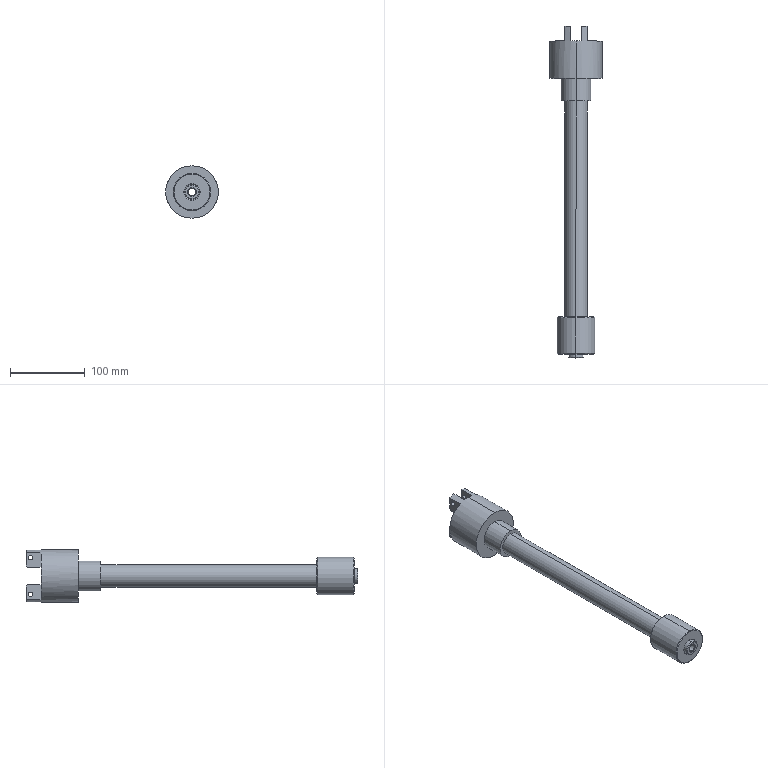Component | SolidWorks | SmallPulley-1 | 2 solids | 68 faces | box 70 x 443.1 x 70 mm | volume 471066 mm3 | cylinder 26 | plane 24 | cone 18 | commonest cylinder face diameters 6 x8 10 x4 20 x4 38.21 x2 70 x2 40 x2 30 x2 50 x2 | material 45
build123d program:
from build123d import *

# Parameters (mm, degrees)
SKETCH1_R           = 25
SKETCH1_R_2         = 10
BOSS_EXTRUDE1_DEPTH = 50
CHAMFER1_SIZE       = 1
SKETCH3_R           = 15
BOSS_EXTRUDE3_DEPTH = 288.1
SKETCH4_R           = 20
BOSS_EXTRUDE4_DEPTH = 30
SKETCH5_R           = 35
BOSS_EXTRUDE5_DEPTH = 70
SKETCH6_R           = 19.105
CUT_EXTRUDE1_DEPTH  = 56.82
CHAMFER3_SIZE       = 2
SKETCH7_R           = 10
BOSS_EXTRUDE6_DEPTH = 55
CHAMFER4_SIZE       = 1
CUT_EXTRUDE2_START  = -20
CUT_EXTRUDE2_DEPTH  = 20
SKETCH10_R          = 3
CUT_EXTRUDE3_DEPTH  = 443.331
SKETCH11_W          = 90
SKETCH11_H          = 14
CUT_EXTRUDE4_DEPTH  = 20
SKETCH12_R          = 5
CUT_EXTRUDE5_DEPTH  = 390.438
CHAMFER5_SIZE       = 1
CHAMFER6_SIZE       = 1


with BuildPart() as part:
    # Sketch1 → Boss-Extrude1 (new body)
    with BuildSketch(Plane.XY):
        Circle(SKETCH1_R)
        Circle(SKETCH1_R_2, mode=Mode.SUBTRACT)
    extrude(amount=BOSS_EXTRUDE1_DEPTH)

    # Chamfer1
    chamfer1_edges = [part.edges().sort_by_distance(p)[0] for p in [
        (-25, 0, 0),
        (-25, 0, 50),
        (-10, 0, 0),
        (-10, 0, 50),
    ]]
    chamfer(chamfer1_edges, length=CHAMFER1_SIZE)

    # Sketch3 → Boss-Extrude3 (add)
    with BuildSketch(Plane(origin=(0, 0, 50), x_dir=(-1, 0, 0), z_dir=(0, 0, -1))):
        Circle(SKETCH3_R)
    extrude(amount=-BOSS_EXTRUDE3_DEPTH)

    # Sketch4 → Boss-Extrude4 (add)
    with BuildSketch(Plane.XY.offset(338.1)):
        Circle(SKETCH4_R)
    extrude(amount=BOSS_EXTRUDE4_DEPTH)

    # Sketch5 → Boss-Extrude5 (add)
    with BuildSketch(Plane.XY.offset(368.1)):
        Circle(SKETCH5_R)
    extrude(amount=BOSS_EXTRUDE5_DEPTH)

    # Sketch6 → Cut-Extrude1 (cut)
    with BuildSketch(Plane.XY.offset(438.1)):
        Circle(SKETCH6_R)
    extrude(amount=-CUT_EXTRUDE1_DEPTH, mode=Mode.SUBTRACT)

    # Chamfer3
    chamfer3_edges = [part.edges().sort_by_distance(p)[0] for p in [
        (-19.105, 0, 438.1),
    ]]
    chamfer(chamfer3_edges, length=CHAMFER3_SIZE)

    # Sketch8 → M5 Tapped Hole1 (revolve, cut)
    with BuildSketch(Plane(origin=(0, 0, 381.28), x_dir=(0, -1, 0), z_dir=(1, 0, 0))):
        Polygon((0, 0), (0, 13.662), (2.1, 12.4), (2.1, 0), align=None)
    revolve(axis=Axis((0, 0, 387.63), (0, 0, -1)), mode=Mode.SUBTRACT)

    # Sketch9 → Cut-Extrude2 (cut)
    with BuildSketch(Plane.XY.offset(438.1).offset(CUT_EXTRUDE2_START)):
        with BuildLine():
            Line((-31.623, 15), (31.623, 15))
            ThreePointArc((31.623, 15), (0, 35), (-31.623, 15))
        make_face()
        with BuildLine():
            Line((-31.623, -15), (31.623, -15))
            ThreePointArc((31.623, -15), (0, -35), (-31.623, -15))
        make_face()
    extrude(amount=CUT_EXTRUDE2_DEPTH, mode=Mode.SUBTRACT)

    # Sketch10 → Cut-Extrude3 (cut, through all)
    with BuildSketch(Plane.XZ.offset(15)):
        with Locations(Location((-24.623, 432.1, 0), (0, 0, 270))):
            Circle(SKETCH10_R)
        with Locations(Location((24.623, 432.1, 0), (0, 0, 270))):
            Circle(SKETCH10_R)
    extrude(amount=-CUT_EXTRUDE3_DEPTH, mode=Mode.SUBTRACT)

    # Sketch11 → Cut-Extrude4 (cut)
    with BuildSketch(Plane.XY.offset(438.1)):
        Rectangle(SKETCH11_W, SKETCH11_H)
    extrude(amount=-CUT_EXTRUDE4_DEPTH, mode=Mode.SUBTRACT)


with BuildPart() as body_2:
    # Sketch7 → Boss-Extrude6 (new body)
    with BuildSketch(Plane(origin=(0, 0, 50), x_dir=(-1, 0, 0), z_dir=(0, 0, -1))):
        with Locations(Location((0, 0, 0), (0, 0, 180))):
            Circle(SKETCH7_R)
    extrude(amount=BOSS_EXTRUDE6_DEPTH)

    # Chamfer4
    chamfer4_edges = [body_2.edges().sort_by_distance(p)[0] for p in [
        (-10, 0, -5),
    ]]
    chamfer(chamfer4_edges, length=CHAMFER4_SIZE)


with BuildPart() as cut_extrude5_tool:
    # Sketch12 → Cut-Extrude5 (new, through all)
    with BuildSketch(Plane.XY.offset(381.28)):
        Circle(SKETCH12_R)
    extrude(amount=-CUT_EXTRUDE5_DEPTH)


with BuildPart() as part_1:
    add(part.part)

    # Cut-Extrude5: cut by cut_extrude5_tool
    add(cut_extrude5_tool.part, mode=Mode.SUBTRACT)

    # Chamfer6
    chamfer6_edges = [part_1.edges().sort_by_distance(p)[0] for p in [
        (-5, 0, 381.28),
    ]]
    chamfer(chamfer6_edges, length=CHAMFER6_SIZE)


with BuildPart() as body_2_1:
    add(body_2.part)

    # Cut-Extrude5: cut by cut_extrude5_tool
    add(cut_extrude5_tool.part, mode=Mode.SUBTRACT)

    # Chamfer5
    chamfer5_edges = [body_2_1.edges().sort_by_distance(p)[0] for p in [
        (-5, 0, -5),
    ]]
    chamfer(chamfer5_edges, length=CHAMFER5_SIZE)


solid = Compound([part_1.part, body_2_1.part])

# Placed as in the assembly
solid = solid.moved(Location((-371.359, -392.185, 1062), (-90, 0, 90)))